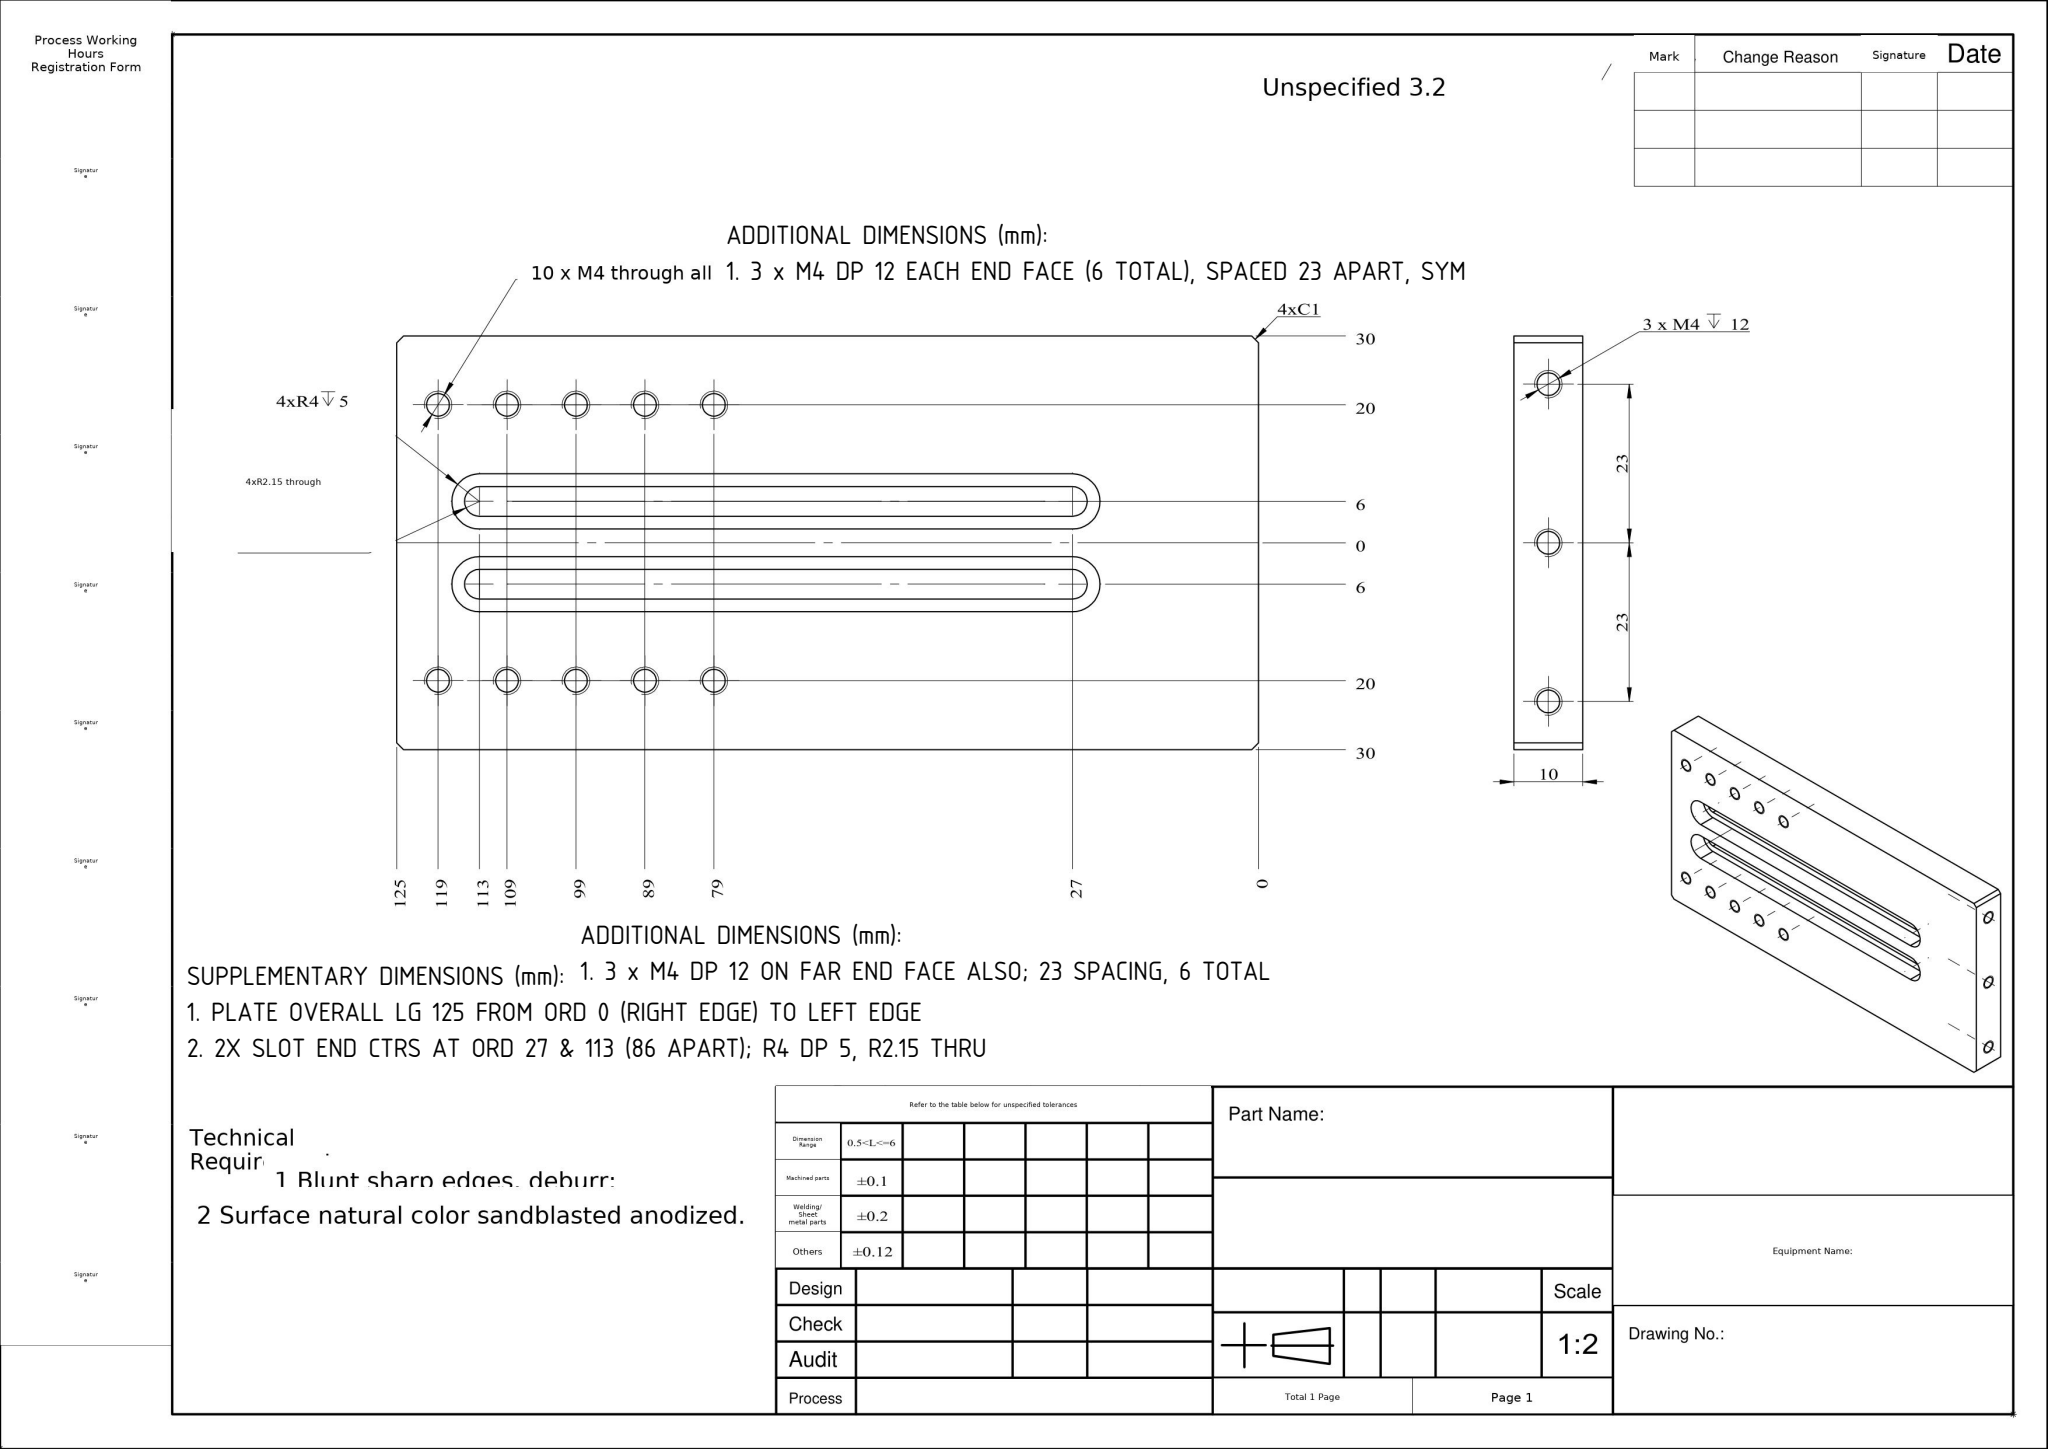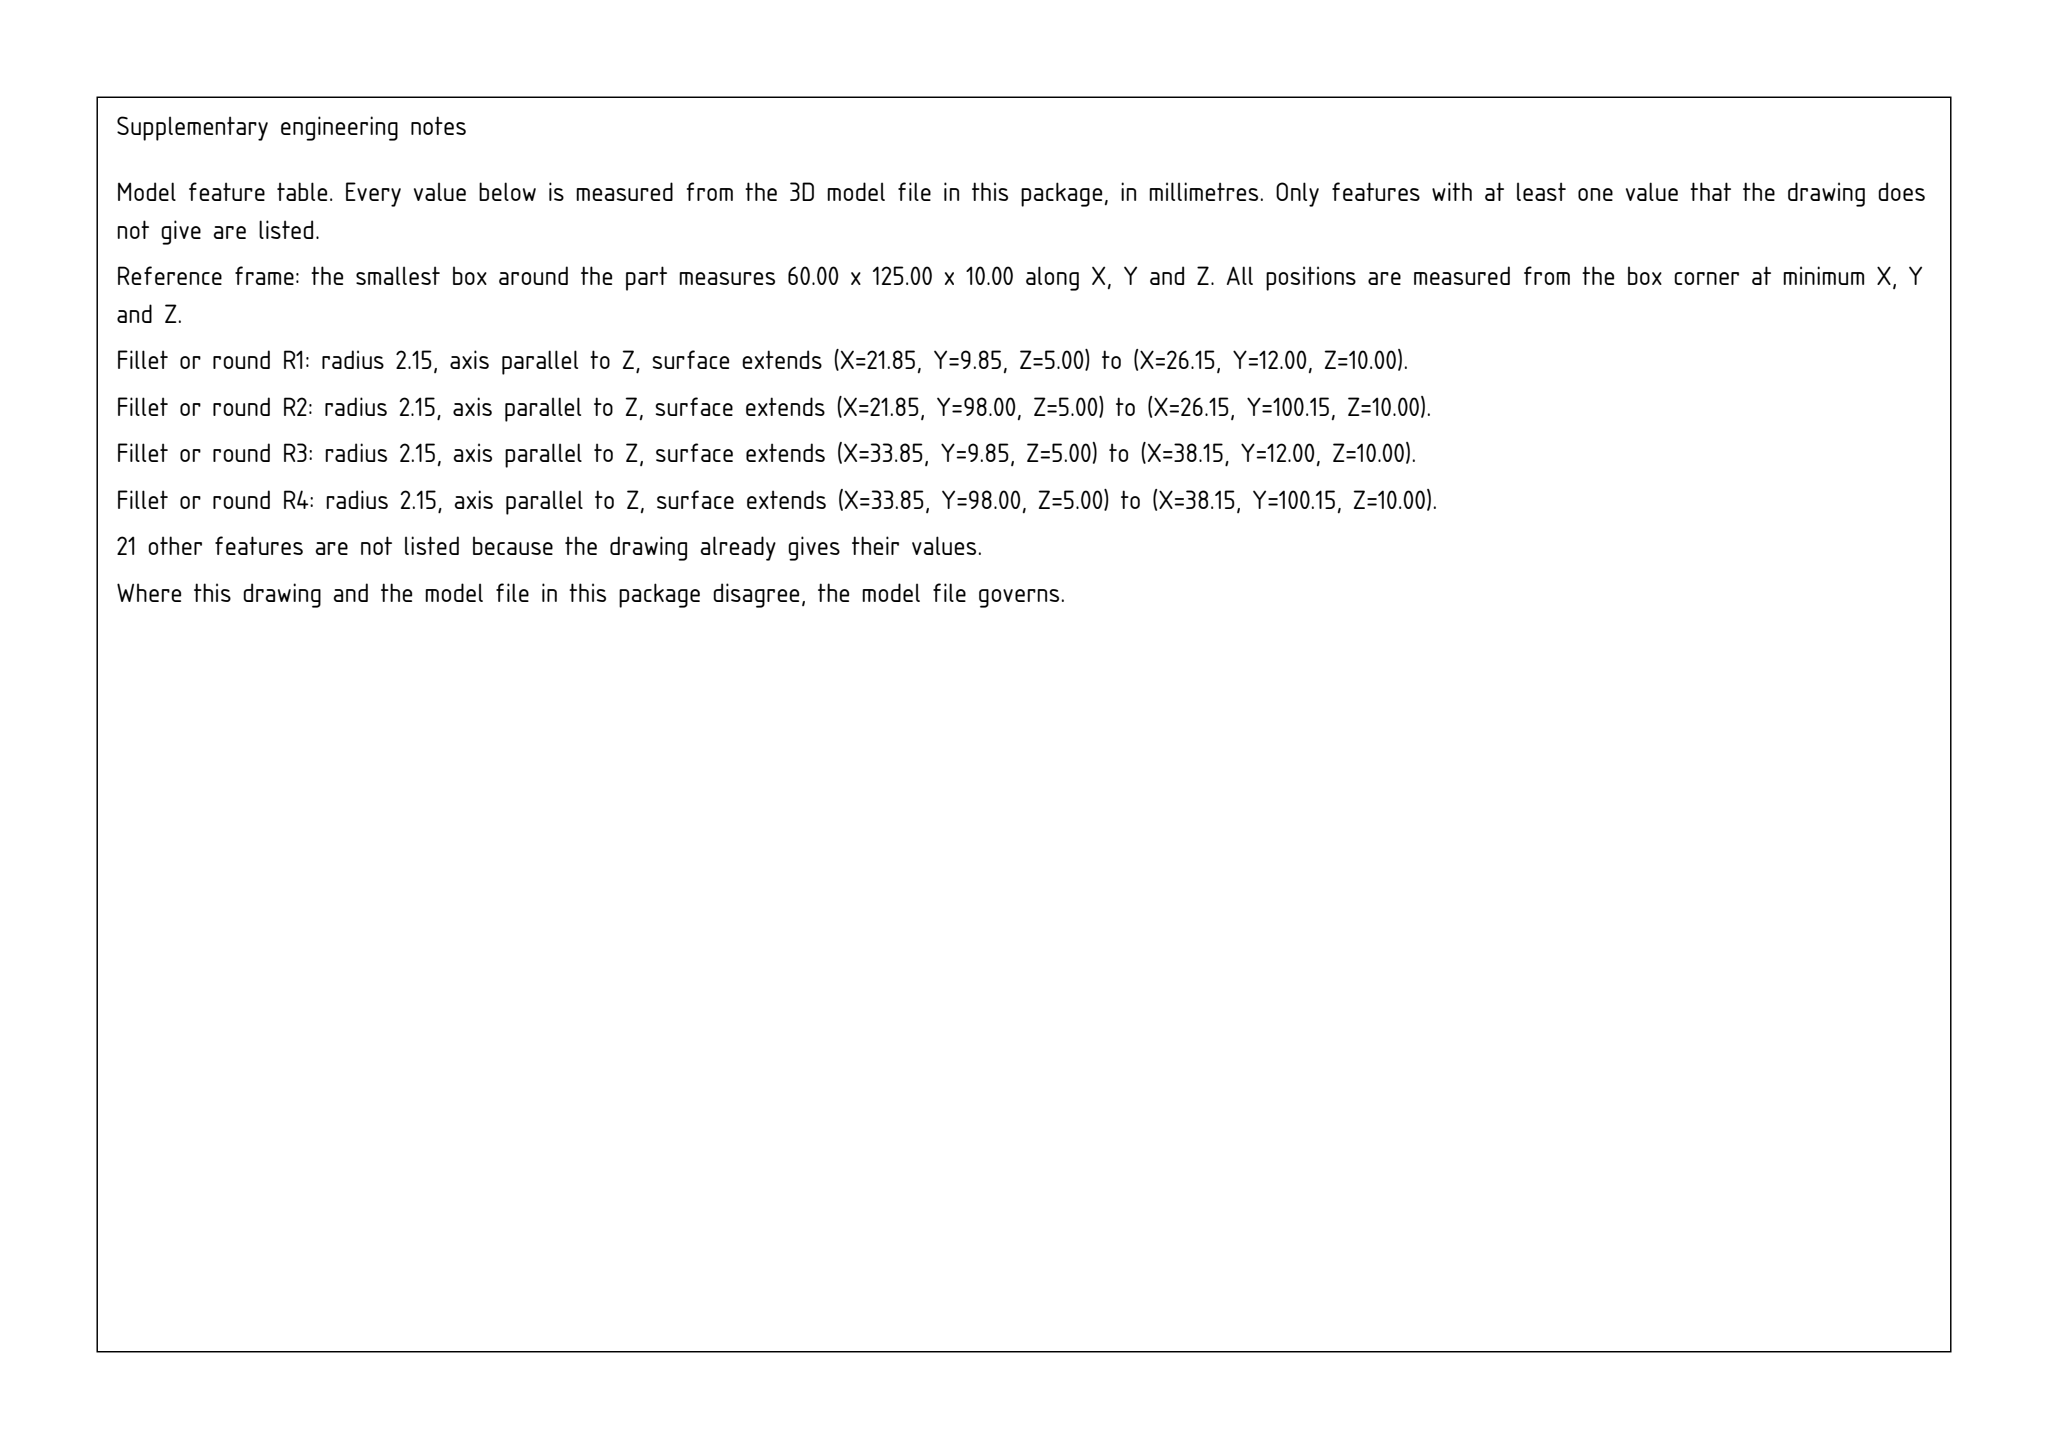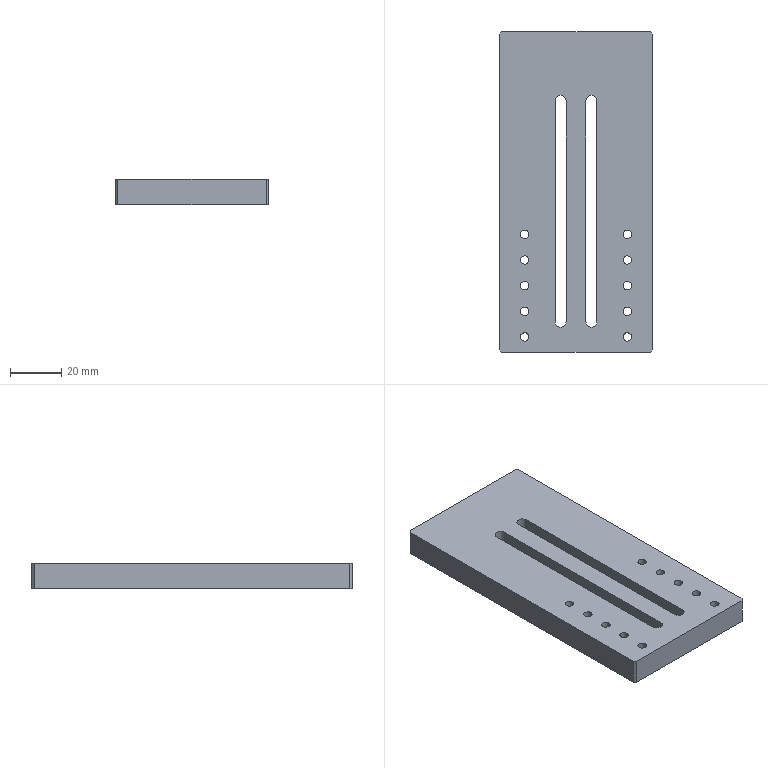Part | SolidWorks | mm | 1 solid | 60 faces | box 60 x 125 x 10 mm | volume 62517 mm3 | cylinder 34 | plane 20 | cone 6 | commonest cylinder face diameters 3.3 x26 4.306 x4 8.006 x4
build123d program:
from build123d import *

# Parameters (mm, degrees)
SKETCH1_W             = 60
SKETCH1_H             = 125
BOSS_EXTRUDE1_DEPTH   = 5
CUT_EXTRUDE1_DEPTH    = 71.045
CUT_EXTRUDE2_DEPTH    = 5
CHAMFER1_SIZE         = 1
M4_TAPPED_HOLE1_D     = 3.3
M4_TAPPED_HOLE2_D     = 3.3
M4_TAPPED_HOLE2_DEPTH = 14.1
M4_TAPPED_HOLE2_TIP   = 0.9914


with BuildPart() as part:
    # Sketch1 → Boss-Extrude1 (new, symmetric)
    with BuildSketch(Plane.XY):
        Rectangle(SKETCH1_W, SKETCH1_H)
    extrude(amount=BOSS_EXTRUDE1_DEPTH, both=True)

    # Sketch2 → Cut-Extrude1 (cut, through all)
    with BuildSketch(Plane.XY.offset(5)):
        with BuildLine():
            Line((-3.847, 35.5), (-3.847, -50.5))
            ThreePointArc((-3.847, -50.5), (-6, -52.653), (-8.153, -50.5))
            Line((-8.153, -50.5), (-8.153, 35.5))
            ThreePointArc((-8.153, 35.5), (-6, 37.653), (-3.847, 35.5))
        make_face()
        with BuildLine():
            Line((8.153, 35.5), (8.153, -50.5))
            ThreePointArc((8.153, -50.5), (6, -52.653), (3.847, -50.5))
            Line((3.847, -50.5), (3.847, 35.5))
            ThreePointArc((3.847, 35.5), (6, 37.653), (8.153, 35.5))
        make_face()
    extrude(amount=-CUT_EXTRUDE1_DEPTH, mode=Mode.SUBTRACT)

    # Sketch3 → Cut-Extrude2 (cut)
    with BuildSketch(Plane.XY.offset(-5)):
        with BuildLine():
            Line((-10.003, 35.5), (-10.003, -50.5))
            ThreePointArc((-10.003, -50.5), (-6, -54.503), (-1.997, -50.5))
            Line((-1.997, -50.5), (-1.997, 35.5))
            ThreePointArc((-1.997, 35.5), (-6, 39.503), (-10.003, 35.5))
        make_face()
        with BuildLine():
            Line((10.003, -50.5), (10.003, 35.5))
            ThreePointArc((10.003, 35.5), (6, 39.503), (1.997, 35.5))
            Line((1.997, 35.5), (1.997, -50.5))
            ThreePointArc((1.997, -50.5), (6, -54.503), (10.003, -50.5))
        make_face()
    extrude(amount=CUT_EXTRUDE2_DEPTH, mode=Mode.SUBTRACT)

    # Chamfer1
    chamfer1_edges = [part.edges().sort_by_distance(p)[0] for p in [
        (30, -62.5, 0),
        (-30, -62.5, 0),
        (-30, 62.5, 0),
        (30, 62.5, 0),
    ]]
    chamfer(chamfer1_edges, length=CHAMFER1_SIZE)

    # M4 Tapped Hole1 (through all)
    with Locations(Plane(origin=(0, 0, -5), x_dir=(-1, 0, 0), z_dir=(0, 0, -1))):
        with Locations((20, -16.5), (-20, -16.5), (-20, -26.5), (-20, -36.5), (-20, -46.5), (-20, -56.5), (20, -26.5), (20, -36.5), (20, -46.5), (20, -56.5)):
            Hole(M4_TAPPED_HOLE1_D / 2)

    # M4 Tapped Hole2
    with Locations(Plane(origin=(0, 62.5, 0), x_dir=(1, 0, 0), z_dir=(0, 1, 0))):
        with Locations((23, 0), (-23, 0), (0, 0)):
            Hole(M4_TAPPED_HOLE2_D / 2, depth=M4_TAPPED_HOLE2_DEPTH)
            with Locations((0, 0, -(M4_TAPPED_HOLE2_DEPTH + M4_TAPPED_HOLE2_TIP / 2))):  # 118° drill point
                Cone(0, M4_TAPPED_HOLE2_D / 2, M4_TAPPED_HOLE2_TIP, mode=Mode.SUBTRACT)


solid = part.part